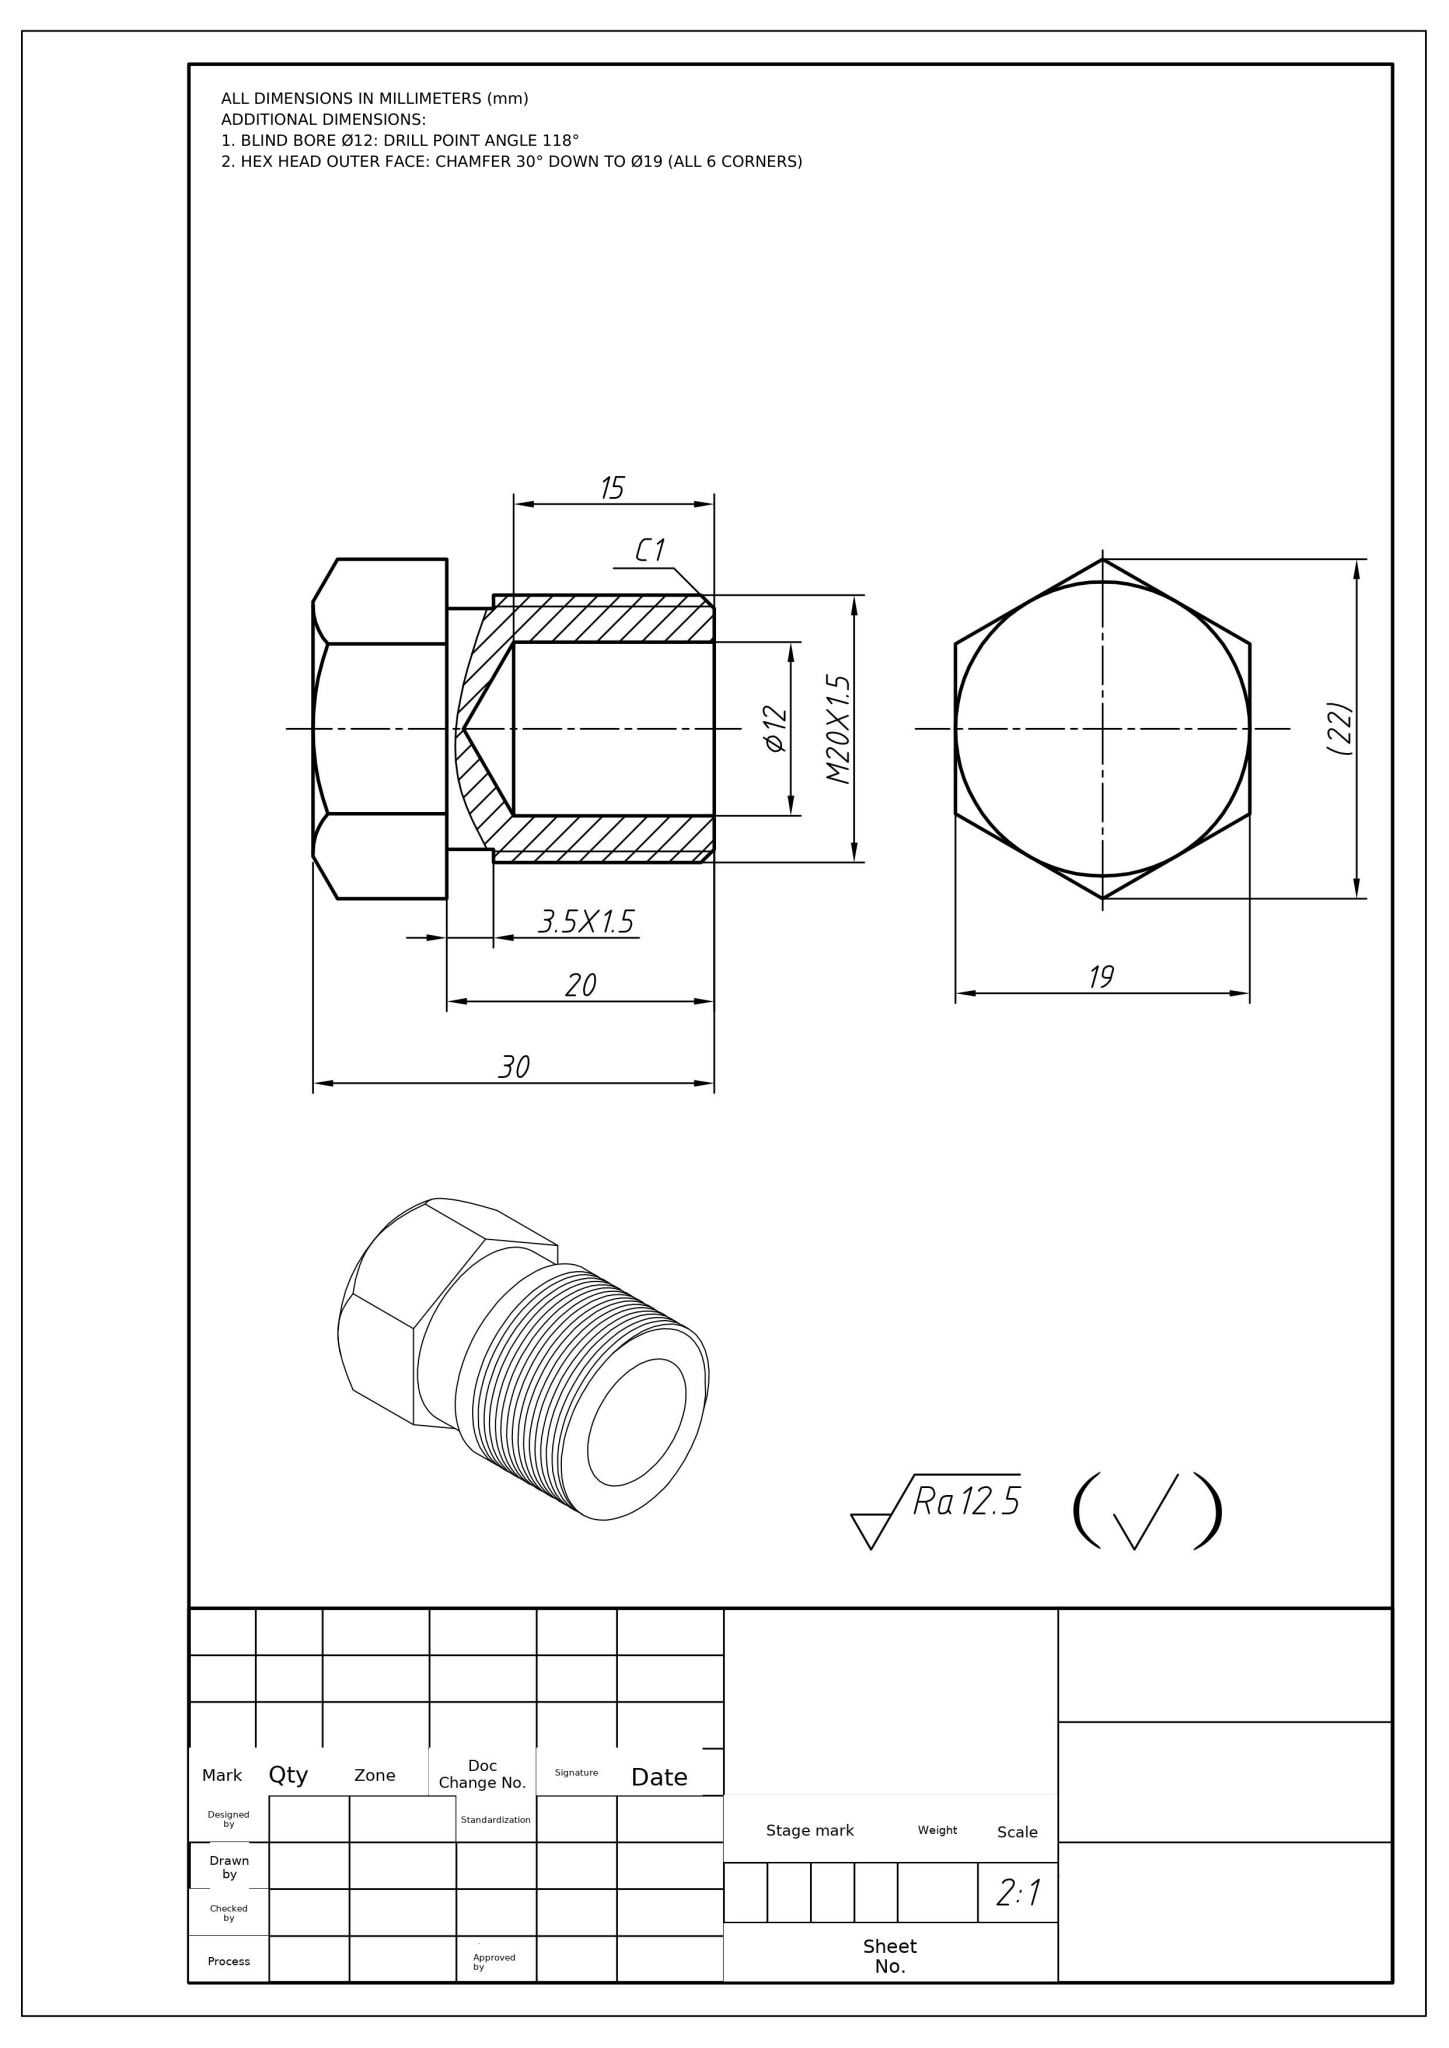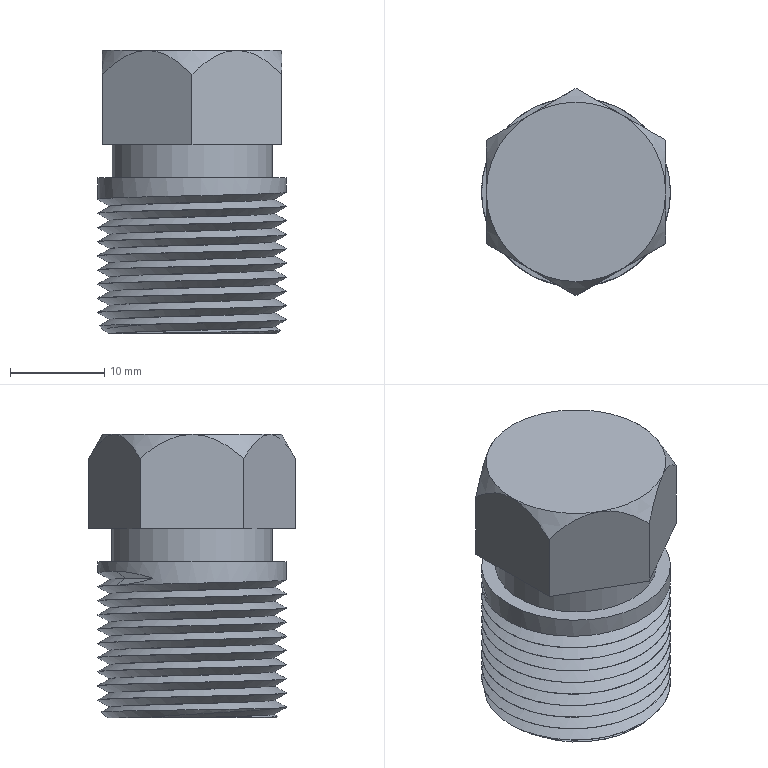Part | NX | mm | 1 solid | 37 faces | box 20 x 21.94 x 30 mm | volume 6651 mm3 | plane 14 | cylinder 13 | cone 8 | spline 2 | commonest cylinder face diameters 20 x10 17 x1 17.5 x1 12 x1